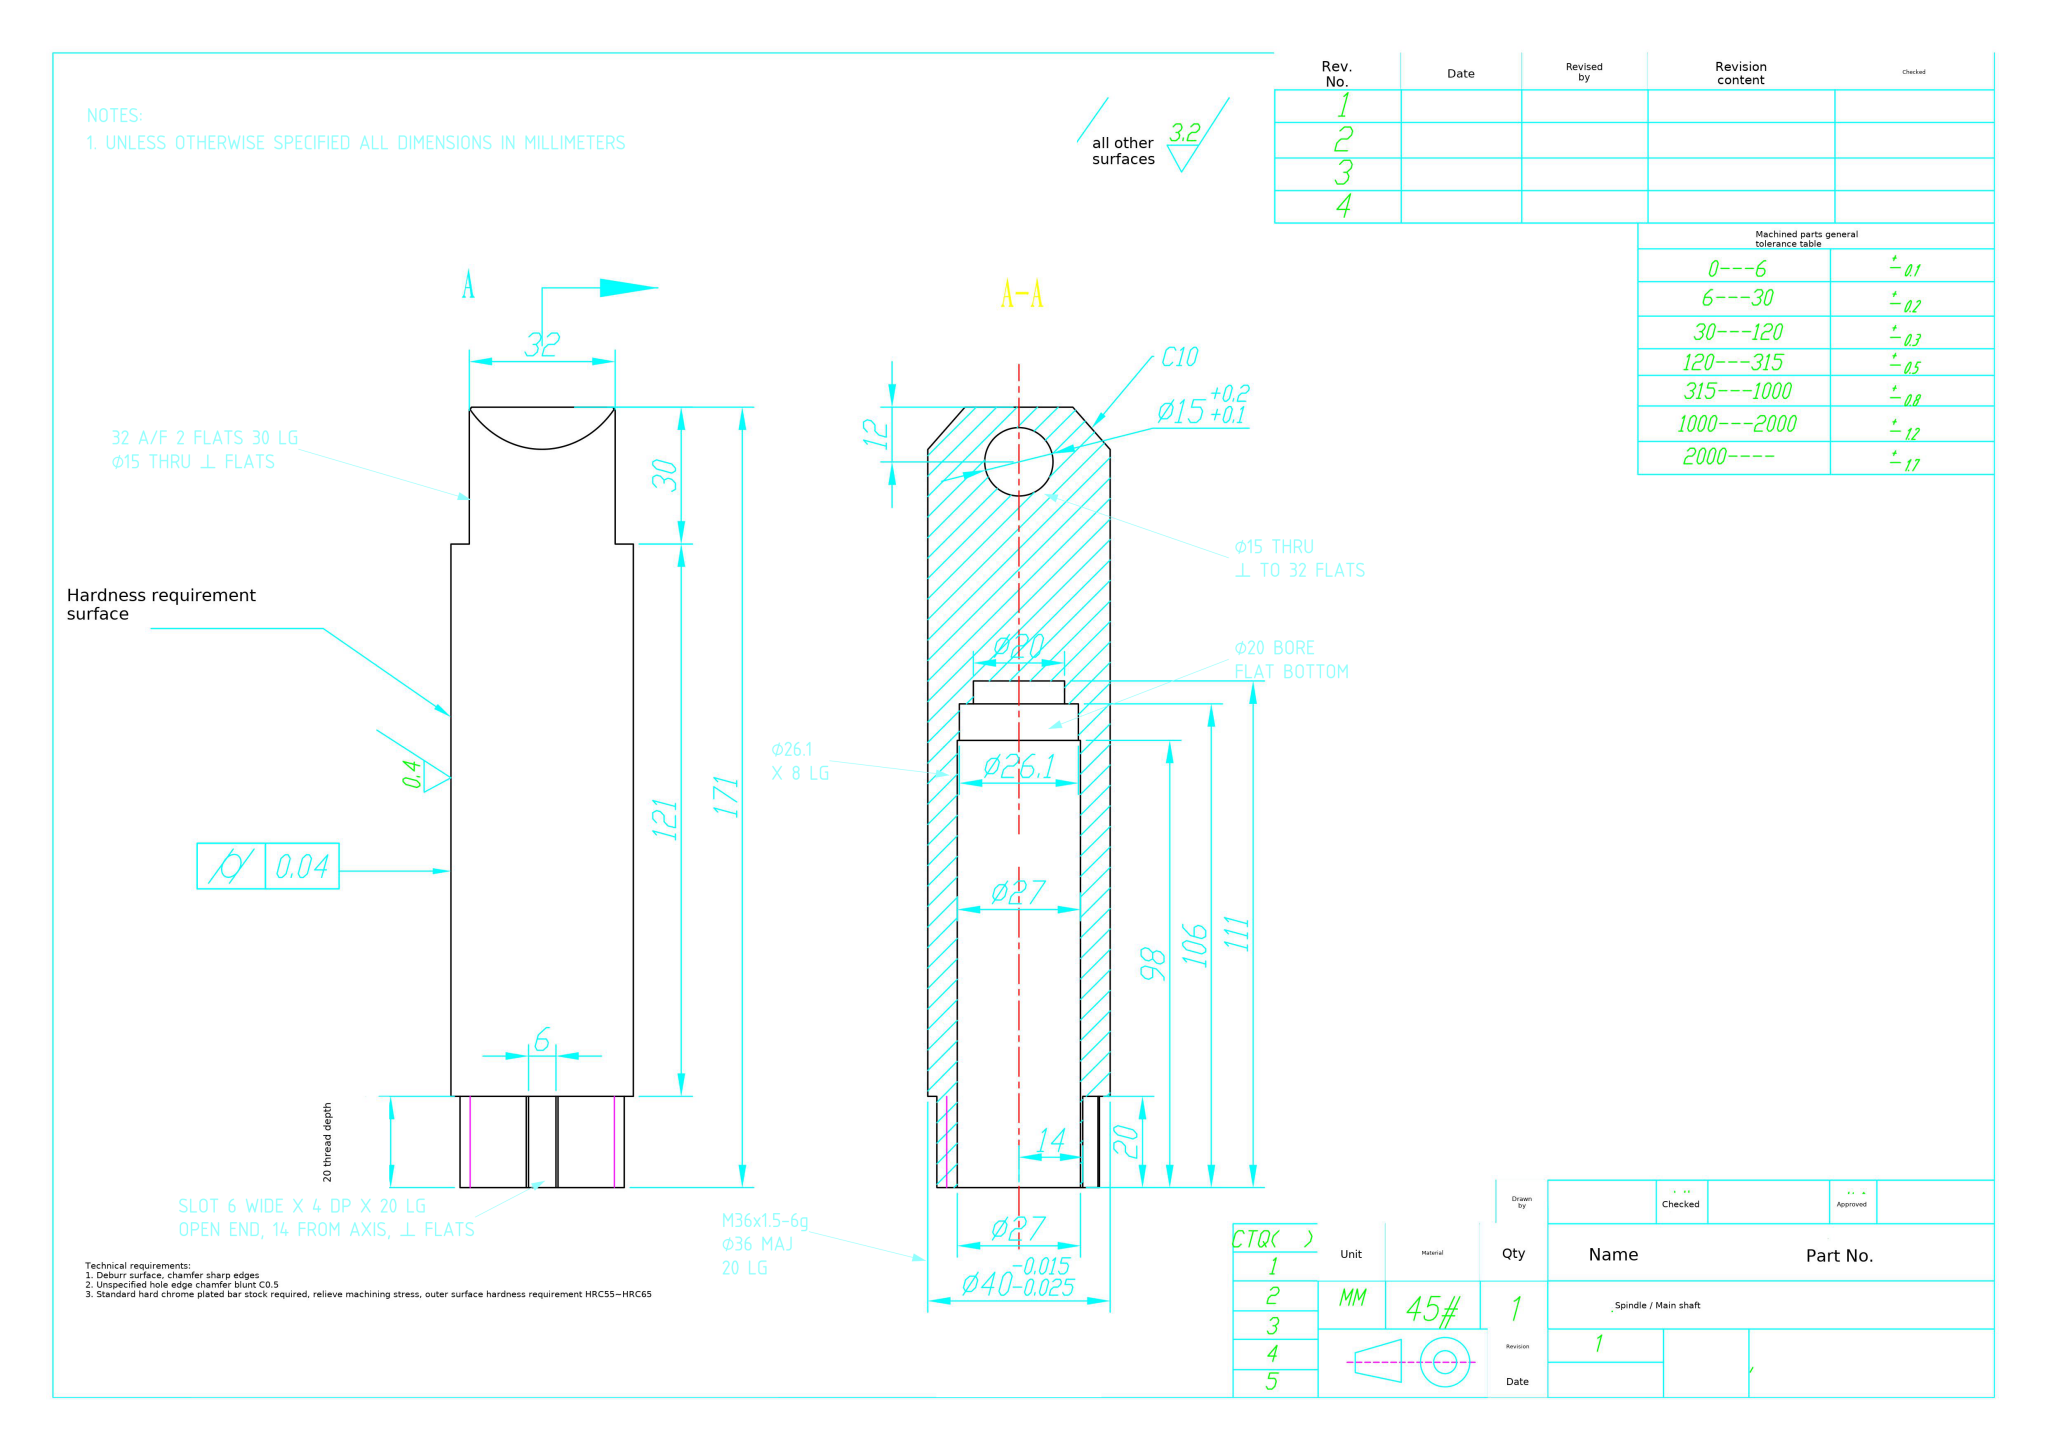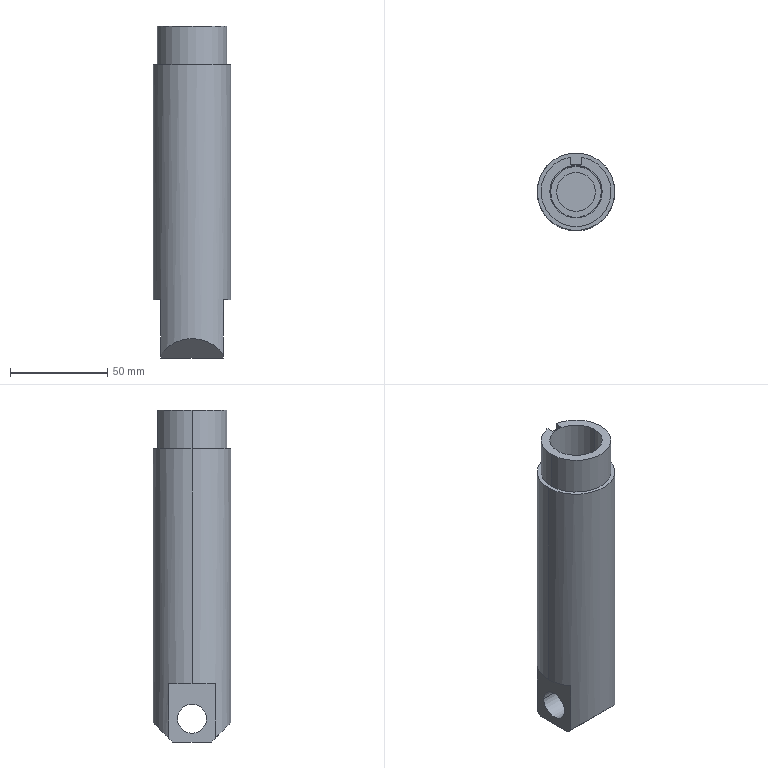Part | NX | mm | 1 solid | 30 faces | box 40 x 40 x 171 mm | volume 136084 mm3 | plane 17 | cylinder 13 | commonest cylinder face diameters 36 x3 40 x2 15 x2 20 x2 26.1 x2 27 x2
STEP:
#1=COLOUR_RGB('',0.7922,0.8196,0.9333);
#2=FILL_AREA_STYLE_COLOUR('',#1);
#3=FILL_AREA_STYLE('',(#2));
#4=SURFACE_STYLE_FILL_AREA(#3);
#5=SURFACE_SIDE_STYLE('',(#4));
#6=SURFACE_STYLE_USAGE(.BOTH.,#5);
#7=PRESENTATION_STYLE_ASSIGNMENT((#6));
#8=CARTESIAN_POINT('',(20.,0.,156.));
#9=VERTEX_POINT('',#8);
#10=CARTESIAN_POINT('',(-20.,0.,156.));
#11=VERTEX_POINT('',#10);
#12=CARTESIAN_POINT('',(0.,0.,156.));
#13=DIRECTION('',(0.,0.,1.));
#14=DIRECTION('',(1.,0.,0.));
#15=AXIS2_PLACEMENT_3D('',#12,#13,#14);
#16=CIRCLE('',#15,20.);
#17=EDGE_CURVE('',#9,#11,#16,.T.);
#18=ORIENTED_EDGE('',*,*,#17,.F.);
#19=CARTESIAN_POINT('',(20.,0.,35.));
#20=VERTEX_POINT('',#19);
#21=CARTESIAN_POINT('',(20.,0.,176.));
#22=DIRECTION('',(0.,0.,-1.));
#23=VECTOR('',#22,1000.);
#24=LINE('',#21,#23);
#25=EDGE_CURVE('',#9,#20,#24,.T.);
#26=ORIENTED_EDGE('',*,*,#25,.T.);
#27=CARTESIAN_POINT('',(16.,12.,35.));
#28=VERTEX_POINT('',#27);
#29=CARTESIAN_POINT('',(0.,0.,35.));
#30=DIRECTION('',(0.,0.,-1.));
#31=DIRECTION('',(-1.,0.,0.));
#32=AXIS2_PLACEMENT_3D('',#29,#30,#31);
#33=CIRCLE('',#32,20.);
#34=EDGE_CURVE('',#28,#20,#33,.T.);
#35=ORIENTED_EDGE('',*,*,#34,.F.);
#36=CARTESIAN_POINT('',(16.,12.,7.));
#37=VERTEX_POINT('',#36);
#38=CARTESIAN_POINT('',(16.,12.,176.));
#39=DIRECTION('',(0.,0.,-1.));
#40=VECTOR('',#39,1000.);
#41=LINE('',#38,#40);
#42=EDGE_CURVE('',#28,#37,#41,.T.);
#43=ORIENTED_EDGE('',*,*,#42,.T.);
#44=CARTESIAN_POINT('',(-16.,12.,7.));
#45=VERTEX_POINT('',#44);
#46=CARTESIAN_POINT('',(16.,12.,7.));
#47=CARTESIAN_POINT('',(7.273,23.636,18.636));
#48=CARTESIAN_POINT('',(-7.273,23.636,18.636));
#49=CARTESIAN_POINT('',(-16.,12.,7.));
#50=(BOUNDED_CURVE()B_SPLINE_CURVE(3,(#46,#47,#48,#49),.UNSPECIFIED.,.F.,.F.)B_SPLINE_CURVE_WITH_KNOTS((4,4),(2.214,4.069),.UNSPECIFIED.)CURVE()GEOMETRIC_REPRESENTATION_ITEM()RATIONAL_B_SPLINE_CURVE((1.,0.7333,0.7333,1.))REPRESENTATION_ITEM(''));
#51=EDGE_CURVE('',#37,#45,#50,.T.);
#52=ORIENTED_EDGE('',*,*,#51,.T.);
#53=CARTESIAN_POINT('',(-16.,12.,35.));
#54=VERTEX_POINT('',#53);
#55=CARTESIAN_POINT('',(-16.,12.,176.));
#56=DIRECTION('',(0.,0.,1.));
#57=VECTOR('',#56,1000.);
#58=LINE('',#55,#57);
#59=EDGE_CURVE('',#45,#54,#58,.T.);
#60=ORIENTED_EDGE('',*,*,#59,.T.);
#61=CARTESIAN_POINT('',(-20.,0.,35.));
#62=VERTEX_POINT('',#61);
#63=CARTESIAN_POINT('',(0.,0.,35.));
#64=DIRECTION('',(0.,0.,-1.));
#65=DIRECTION('',(-1.,0.,0.));
#66=AXIS2_PLACEMENT_3D('',#63,#64,#65);
#67=CIRCLE('',#66,20.);
#68=EDGE_CURVE('',#62,#54,#67,.T.);
#69=ORIENTED_EDGE('',*,*,#68,.F.);
#70=CARTESIAN_POINT('',(-20.,0.,176.));
#71=DIRECTION('',(0.,0.,-1.));
#72=VECTOR('',#71,1000.);
#73=LINE('',#70,#72);
#74=EDGE_CURVE('',#11,#62,#73,.T.);
#75=ORIENTED_EDGE('',*,*,#74,.F.);
#76=EDGE_LOOP('',(#18,#26,#35,#43,#52,#60,#69,#75));
#77=FACE_OUTER_BOUND('',#76,.T.);
#78=CARTESIAN_POINT('',(0.,0.,176.));
#79=DIRECTION('',(0.,0.,-1.));
#80=DIRECTION('',(-1.,0.,0.));
#81=AXIS2_PLACEMENT_3D('',#78,#79,#80);
#82=CYLINDRICAL_SURFACE('',#81,20.);
#83=ADVANCED_FACE('',(#77),#82,.T.);
#84=CARTESIAN_POINT('',(16.,7.5,17.));
#85=VERTEX_POINT('',#84);
#86=CARTESIAN_POINT('',(16.,-7.5,17.));
#87=VERTEX_POINT('',#86);
#88=CARTESIAN_POINT('',(16.,-0.,17.));
#89=DIRECTION('',(-1.,0.,0.));
#90=DIRECTION('',(0.,-1.,0.));
#91=AXIS2_PLACEMENT_3D('',#88,#89,#90);
#92=CIRCLE('',#91,7.5);
#93=EDGE_CURVE('',#85,#87,#92,.T.);
#94=ORIENTED_EDGE('',*,*,#93,.F.);
#95=CARTESIAN_POINT('',(-16.,7.5,17.));
#96=VERTEX_POINT('',#95);
#97=CARTESIAN_POINT('',(20.,7.5,17.));
#98=DIRECTION('',(-1.,0.,0.));
#99=VECTOR('',#98,1000.);
#100=LINE('',#97,#99);
#101=EDGE_CURVE('',#85,#96,#100,.T.);
#102=ORIENTED_EDGE('',*,*,#101,.T.);
#103=CARTESIAN_POINT('',(-16.,-7.5,17.));
#104=VERTEX_POINT('',#103);
#105=CARTESIAN_POINT('',(-16.,0.,17.));
#106=DIRECTION('',(-1.,0.,0.));
#107=DIRECTION('',(0.,-1.,0.));
#108=AXIS2_PLACEMENT_3D('',#105,#106,#107);
#109=CIRCLE('',#108,7.5);
#110=EDGE_CURVE('',#96,#104,#109,.T.);
#111=ORIENTED_EDGE('',*,*,#110,.T.);
#112=CARTESIAN_POINT('',(20.,-7.5,17.));
#113=DIRECTION('',(-1.,0.,0.));
#114=VECTOR('',#113,1000.);
#115=LINE('',#112,#114);
#116=EDGE_CURVE('',#87,#104,#115,.T.);
#117=ORIENTED_EDGE('',*,*,#116,.F.);
#118=EDGE_LOOP('',(#94,#102,#111,#117));
#119=FACE_OUTER_BOUND('',#118,.T.);
#120=CARTESIAN_POINT('',(20.,-0.,17.));
#121=DIRECTION('',(-1.,0.,0.));
#122=DIRECTION('',(0.,-1.,0.));
#123=AXIS2_PLACEMENT_3D('',#120,#121,#122);
#124=CYLINDRICAL_SURFACE('',#123,7.5);
#125=ADVANCED_FACE('',(#119),#124,.F.);
#126=CARTESIAN_POINT('',(-3.485,17.659,156.));
#127=VERTEX_POINT('',#126);
#128=CARTESIAN_POINT('',(-18.,0.,156.));
#129=VERTEX_POINT('',#128);
#130=CARTESIAN_POINT('',(0.,0.,156.));
#131=DIRECTION('',(0.,0.,1.));
#132=DIRECTION('',(1.,0.,0.));
#133=AXIS2_PLACEMENT_3D('',#130,#131,#132);
#134=CIRCLE('',#133,18.);
#135=EDGE_CURVE('',#127,#129,#134,.T.);
#136=ORIENTED_EDGE('',*,*,#135,.T.);
#137=CARTESIAN_POINT('',(-18.,0.,176.));
#138=VERTEX_POINT('',#137);
#139=CARTESIAN_POINT('',(-18.,0.,156.));
#140=DIRECTION('',(0.,0.,1.));
#141=VECTOR('',#140,1000.);
#142=LINE('',#139,#141);
#143=EDGE_CURVE('',#129,#138,#142,.T.);
#144=ORIENTED_EDGE('',*,*,#143,.T.);
#145=CARTESIAN_POINT('',(-3.485,17.659,176.));
#146=VERTEX_POINT('',#145);
#147=CARTESIAN_POINT('',(0.,0.,176.));
#148=DIRECTION('',(0.,0.,1.));
#149=DIRECTION('',(1.,0.,0.));
#150=AXIS2_PLACEMENT_3D('',#147,#148,#149);
#151=CIRCLE('',#150,18.);
#152=EDGE_CURVE('',#146,#138,#151,.T.);
#153=ORIENTED_EDGE('',*,*,#152,.F.);
#154=CARTESIAN_POINT('',(-3.485,17.659,156.));
#155=DIRECTION('',(0.,0.,-1.));
#156=VECTOR('',#155,1000.);
#157=LINE('',#154,#156);
#158=EDGE_CURVE('',#146,#127,#157,.T.);
#159=ORIENTED_EDGE('',*,*,#158,.T.);
#160=EDGE_LOOP('',(#136,#144,#153,#159));
#161=FACE_OUTER_BOUND('',#160,.T.);
#162=CARTESIAN_POINT('',(0.,0.,156.));
#163=DIRECTION('',(0.,0.,1.));
#164=DIRECTION('',(1.,0.,0.));
#165=AXIS2_PLACEMENT_3D('',#162,#163,#164);
#166=CYLINDRICAL_SURFACE('',#165,18.);
#167=ADVANCED_FACE('',(#161),#166,.T.);
#168=ORIENTED_EDGE('',*,*,#143,.F.);
#169=CARTESIAN_POINT('',(18.,0.,156.));
#170=VERTEX_POINT('',#169);
#171=CARTESIAN_POINT('',(0.,0.,156.));
#172=DIRECTION('',(0.,0.,1.));
#173=DIRECTION('',(1.,0.,0.));
#174=AXIS2_PLACEMENT_3D('',#171,#172,#173);
#175=CIRCLE('',#174,18.);
#176=EDGE_CURVE('',#129,#170,#175,.T.);
#177=ORIENTED_EDGE('',*,*,#176,.T.);
#178=CARTESIAN_POINT('',(18.,0.,176.));
#179=VERTEX_POINT('',#178);
#180=CARTESIAN_POINT('',(18.,0.,156.));
#181=DIRECTION('',(0.,0.,1.));
#182=VECTOR('',#181,1000.);
#183=LINE('',#180,#182);
#184=EDGE_CURVE('',#170,#179,#183,.T.);
#185=ORIENTED_EDGE('',*,*,#184,.T.);
#186=CARTESIAN_POINT('',(0.,0.,176.));
#187=DIRECTION('',(0.,0.,1.));
#188=DIRECTION('',(1.,0.,0.));
#189=AXIS2_PLACEMENT_3D('',#186,#187,#188);
#190=CIRCLE('',#189,18.);
#191=EDGE_CURVE('',#138,#179,#190,.T.);
#192=ORIENTED_EDGE('',*,*,#191,.F.);
#193=EDGE_LOOP('',(#168,#177,#185,#192));
#194=FACE_OUTER_BOUND('',#193,.T.);
#195=CARTESIAN_POINT('',(0.,0.,156.));
#196=DIRECTION('',(0.,0.,1.));
#197=DIRECTION('',(1.,0.,0.));
#198=AXIS2_PLACEMENT_3D('',#195,#196,#197);
#199=CYLINDRICAL_SURFACE('',#198,18.);
#200=ADVANCED_FACE('',(#194),#199,.T.);
#201=CARTESIAN_POINT('',(-10.,0.,65.));
#202=VERTEX_POINT('',#201);
#203=CARTESIAN_POINT('',(10.,0.,65.));
#204=VERTEX_POINT('',#203);
#205=CARTESIAN_POINT('',(0.,0.,65.));
#206=DIRECTION('',(0.,0.,1.));
#207=DIRECTION('',(1.,0.,0.));
#208=AXIS2_PLACEMENT_3D('',#205,#206,#207);
#209=CIRCLE('',#208,10.);
#210=EDGE_CURVE('',#202,#204,#209,.T.);
#211=ORIENTED_EDGE('',*,*,#210,.F.);
#212=CARTESIAN_POINT('',(-10.,0.,70.));
#213=VERTEX_POINT('',#212);
#214=CARTESIAN_POINT('',(-10.,0.,65.));
#215=DIRECTION('',(0.,0.,1.));
#216=VECTOR('',#215,1000.);
#217=LINE('',#214,#216);
#218=EDGE_CURVE('',#202,#213,#217,.T.);
#219=ORIENTED_EDGE('',*,*,#218,.T.);
#220=CARTESIAN_POINT('',(10.,0.,70.));
#221=VERTEX_POINT('',#220);
#222=CARTESIAN_POINT('',(0.,0.,70.));
#223=DIRECTION('',(0.,0.,1.));
#224=DIRECTION('',(1.,0.,0.));
#225=AXIS2_PLACEMENT_3D('',#222,#223,#224);
#226=CIRCLE('',#225,10.);
#227=EDGE_CURVE('',#213,#221,#226,.T.);
#228=ORIENTED_EDGE('',*,*,#227,.T.);
#229=CARTESIAN_POINT('',(10.,0.,65.));
#230=DIRECTION('',(0.,0.,1.));
#231=VECTOR('',#230,1000.);
#232=LINE('',#229,#231);
#233=EDGE_CURVE('',#204,#221,#232,.T.);
#234=ORIENTED_EDGE('',*,*,#233,.F.);
#235=EDGE_LOOP('',(#211,#219,#228,#234));
#236=FACE_OUTER_BOUND('',#235,.T.);
#237=CARTESIAN_POINT('',(0.,0.,65.));
#238=DIRECTION('',(0.,0.,1.));
#239=DIRECTION('',(1.,0.,0.));
#240=AXIS2_PLACEMENT_3D('',#237,#238,#239);
#241=CYLINDRICAL_SURFACE('',#240,10.);
#242=ADVANCED_FACE('',(#236),#241,.F.);
#243=CARTESIAN_POINT('',(-13.05,0.,70.));
#244=VERTEX_POINT('',#243);
#245=CARTESIAN_POINT('',(13.05,0.,70.));
#246=VERTEX_POINT('',#245);
#247=CARTESIAN_POINT('',(0.,0.,70.));
#248=DIRECTION('',(0.,0.,1.));
#249=DIRECTION('',(1.,0.,0.));
#250=AXIS2_PLACEMENT_3D('',#247,#248,#249);
#251=CIRCLE('',#250,13.05);
#252=EDGE_CURVE('',#244,#246,#251,.T.);
#253=ORIENTED_EDGE('',*,*,#252,.F.);
#254=CARTESIAN_POINT('',(-13.05,0.,78.));
#255=VERTEX_POINT('',#254);
#256=CARTESIAN_POINT('',(-13.05,0.,70.));
#257=DIRECTION('',(0.,0.,1.));
#258=VECTOR('',#257,1000.);
#259=LINE('',#256,#258);
#260=EDGE_CURVE('',#244,#255,#259,.T.);
#261=ORIENTED_EDGE('',*,*,#260,.T.);
#262=CARTESIAN_POINT('',(13.05,0.,78.));
#263=VERTEX_POINT('',#262);
#264=CARTESIAN_POINT('',(0.,0.,78.));
#265=DIRECTION('',(0.,0.,1.));
#266=DIRECTION('',(1.,0.,0.));
#267=AXIS2_PLACEMENT_3D('',#264,#265,#266);
#268=CIRCLE('',#267,13.05);
#269=EDGE_CURVE('',#255,#263,#268,.T.);
#270=ORIENTED_EDGE('',*,*,#269,.T.);
#271=CARTESIAN_POINT('',(13.05,0.,70.));
#272=DIRECTION('',(0.,0.,1.));
#273=VECTOR('',#272,1000.);
#274=LINE('',#271,#273);
#275=EDGE_CURVE('',#246,#263,#274,.T.);
#276=ORIENTED_EDGE('',*,*,#275,.F.);
#277=EDGE_LOOP('',(#253,#261,#270,#276));
#278=FACE_OUTER_BOUND('',#277,.T.);
#279=CARTESIAN_POINT('',(0.,0.,70.));
#280=DIRECTION('',(0.,0.,1.));
#281=DIRECTION('',(1.,0.,0.));
#282=AXIS2_PLACEMENT_3D('',#279,#280,#281);
#283=CYLINDRICAL_SURFACE('',#282,13.05);
#284=ADVANCED_FACE('',(#278),#283,.F.);
#285=CARTESIAN_POINT('',(-13.5,0.,78.));
#286=VERTEX_POINT('',#285);
#287=CARTESIAN_POINT('',(13.5,0.,78.));
#288=VERTEX_POINT('',#287);
#289=CARTESIAN_POINT('',(0.,0.,78.));
#290=DIRECTION('',(0.,0.,1.));
#291=DIRECTION('',(1.,0.,0.));
#292=AXIS2_PLACEMENT_3D('',#289,#290,#291);
#293=CIRCLE('',#292,13.5);
#294=EDGE_CURVE('',#286,#288,#293,.T.);
#295=ORIENTED_EDGE('',*,*,#294,.F.);
#296=CARTESIAN_POINT('',(-13.5,0.,176.));
#297=VERTEX_POINT('',#296);
#298=CARTESIAN_POINT('',(-13.5,0.,78.));
#299=DIRECTION('',(0.,0.,1.));
#300=VECTOR('',#299,1000.);
#301=LINE('',#298,#300);
#302=EDGE_CURVE('',#286,#297,#301,.T.);
#303=ORIENTED_EDGE('',*,*,#302,.T.);
#304=CARTESIAN_POINT('',(13.5,0.,176.));
#305=VERTEX_POINT('',#304);
#306=CARTESIAN_POINT('',(0.,0.,176.));
#307=DIRECTION('',(0.,0.,1.));
#308=DIRECTION('',(1.,0.,0.));
#309=AXIS2_PLACEMENT_3D('',#306,#307,#308);
#310=CIRCLE('',#309,13.5);
#311=EDGE_CURVE('',#297,#305,#310,.T.);
#312=ORIENTED_EDGE('',*,*,#311,.T.);
#313=CARTESIAN_POINT('',(13.5,0.,78.));
#314=DIRECTION('',(0.,0.,1.));
#315=VECTOR('',#314,1000.);
#316=LINE('',#313,#315);
#317=EDGE_CURVE('',#288,#305,#316,.T.);
#318=ORIENTED_EDGE('',*,*,#317,.F.);
#319=EDGE_LOOP('',(#295,#303,#312,#318));
#320=FACE_OUTER_BOUND('',#319,.T.);
#321=CARTESIAN_POINT('',(0.,0.,78.));
#322=DIRECTION('',(0.,0.,1.));
#323=DIRECTION('',(1.,0.,0.));
#324=AXIS2_PLACEMENT_3D('',#321,#322,#323);
#325=CYLINDRICAL_SURFACE('',#324,13.5);
#326=ADVANCED_FACE('',(#320),#325,.F.);
#327=ORIENTED_EDGE('',*,*,#152,.T.);
#328=ORIENTED_EDGE('',*,*,#191,.T.);
#329=CARTESIAN_POINT('',(3.485,17.659,176.));
#330=VERTEX_POINT('',#329);
#331=CARTESIAN_POINT('',(0.,0.,176.));
#332=DIRECTION('',(0.,0.,1.));
#333=DIRECTION('',(1.,0.,0.));
#334=AXIS2_PLACEMENT_3D('',#331,#332,#333);
#335=CIRCLE('',#334,18.);
#336=EDGE_CURVE('',#179,#330,#335,.T.);
#337=ORIENTED_EDGE('',*,*,#336,.T.);
#338=CARTESIAN_POINT('',(3.,17.314,176.));
#339=VERTEX_POINT('',#338);
#340=CARTESIAN_POINT('',(-7.169,10.086,176.));
#341=DIRECTION('',(-0.8151,-0.5794,0.));
#342=VECTOR('',#341,1000.);
#343=LINE('',#340,#342);
#344=EDGE_CURVE('',#330,#339,#343,.T.);
#345=ORIENTED_EDGE('',*,*,#344,.T.);
#346=CARTESIAN_POINT('',(3.,14.,176.));
#347=VERTEX_POINT('',#346);
#348=CARTESIAN_POINT('',(3.,18.886,176.));
#349=DIRECTION('',(-0.,1.,0.));
#350=VECTOR('',#349,1000.);
#351=LINE('',#348,#350);
#352=EDGE_CURVE('',#347,#339,#351,.T.);
#353=ORIENTED_EDGE('',*,*,#352,.F.);
#354=CARTESIAN_POINT('',(-3.,14.,176.));
#355=VERTEX_POINT('',#354);
#356=CARTESIAN_POINT('',(-3.,14.,176.));
#357=DIRECTION('',(1.,0.,0.));
#358=VECTOR('',#357,1000.);
#359=LINE('',#356,#358);
#360=EDGE_CURVE('',#355,#347,#359,.T.);
#361=ORIENTED_EDGE('',*,*,#360,.F.);
#362=CARTESIAN_POINT('',(-3.,17.314,176.));
#363=VERTEX_POINT('',#362);
#364=CARTESIAN_POINT('',(-3.,18.886,176.));
#365=DIRECTION('',(0.,-1.,0.));
#366=VECTOR('',#365,1000.);
#367=LINE('',#364,#366);
#368=EDGE_CURVE('',#363,#355,#367,.T.);
#369=ORIENTED_EDGE('',*,*,#368,.F.);
#370=CARTESIAN_POINT('',(7.169,10.086,176.));
#371=DIRECTION('',(-0.8151,0.5794,0.));
#372=VECTOR('',#371,1000.);
#373=LINE('',#370,#372);
#374=EDGE_CURVE('',#363,#146,#373,.T.);
#375=ORIENTED_EDGE('',*,*,#374,.T.);
#376=EDGE_LOOP('',(#327,#328,#337,#345,#353,#361,#369,#375));
#377=FACE_OUTER_BOUND('',#376,.T.);
#378=CARTESIAN_POINT('',(0.,0.,176.));
#379=DIRECTION('',(0.,0.,1.));
#380=DIRECTION('',(1.,0.,0.));
#381=AXIS2_PLACEMENT_3D('',#378,#379,#380);
#382=CIRCLE('',#381,13.5);
#383=EDGE_CURVE('',#305,#297,#382,.T.);
#384=ORIENTED_EDGE('',*,*,#383,.F.);
#385=ORIENTED_EDGE('',*,*,#311,.F.);
#386=EDGE_LOOP('',(#384,#385));
#387=FACE_BOUND('',#386,.T.);
#388=CARTESIAN_POINT('',(0.,0.,176.));
#389=DIRECTION('',(0.,0.,1.));
#390=DIRECTION('',(1.,0.,0.));
#391=AXIS2_PLACEMENT_3D('',#388,#389,#390);
#392=PLANE('',#391);
#393=ADVANCED_FACE('',(#377,#387),#392,.T.);
#394=ORIENTED_EDGE('',*,*,#302,.F.);
#395=CARTESIAN_POINT('',(0.,0.,78.));
#396=DIRECTION('',(0.,0.,1.));
#397=DIRECTION('',(1.,0.,0.));
#398=AXIS2_PLACEMENT_3D('',#395,#396,#397);
#399=CIRCLE('',#398,13.5);
#400=EDGE_CURVE('',#288,#286,#399,.T.);
#401=ORIENTED_EDGE('',*,*,#400,.F.);
#402=ORIENTED_EDGE('',*,*,#317,.T.);
#403=ORIENTED_EDGE('',*,*,#383,.T.);
#404=EDGE_LOOP('',(#394,#401,#402,#403));
#405=FACE_OUTER_BOUND('',#404,.T.);
#406=CARTESIAN_POINT('',(0.,0.,78.));
#407=DIRECTION('',(0.,0.,1.));
#408=DIRECTION('',(1.,0.,0.));
#409=AXIS2_PLACEMENT_3D('',#406,#407,#408);
#410=CYLINDRICAL_SURFACE('',#409,13.5);
#411=ADVANCED_FACE('',(#405),#410,.F.);
#412=CARTESIAN_POINT('',(0.,0.,78.));
#413=DIRECTION('',(0.,0.,1.));
#414=DIRECTION('',(1.,0.,0.));
#415=AXIS2_PLACEMENT_3D('',#412,#413,#414);
#416=CIRCLE('',#415,13.05);
#417=EDGE_CURVE('',#263,#255,#416,.T.);
#418=ORIENTED_EDGE('',*,*,#417,.F.);
#419=ORIENTED_EDGE('',*,*,#269,.F.);
#420=EDGE_LOOP('',(#418,#419));
#421=FACE_BOUND('',#420,.T.);
#422=ORIENTED_EDGE('',*,*,#400,.T.);
#423=ORIENTED_EDGE('',*,*,#294,.T.);
#424=EDGE_LOOP('',(#422,#423));
#425=FACE_OUTER_BOUND('',#424,.T.);
#426=CARTESIAN_POINT('',(0.,0.,78.));
#427=DIRECTION('',(0.,0.,1.));
#428=DIRECTION('',(1.,0.,0.));
#429=AXIS2_PLACEMENT_3D('',#426,#427,#428);
#430=PLANE('',#429);
#431=ADVANCED_FACE('',(#421,#425),#430,.T.);
#432=ORIENTED_EDGE('',*,*,#260,.F.);
#433=CARTESIAN_POINT('',(0.,0.,70.));
#434=DIRECTION('',(0.,0.,1.));
#435=DIRECTION('',(1.,0.,0.));
#436=AXIS2_PLACEMENT_3D('',#433,#434,#435);
#437=CIRCLE('',#436,13.05);
#438=EDGE_CURVE('',#246,#244,#437,.T.);
#439=ORIENTED_EDGE('',*,*,#438,.F.);
#440=ORIENTED_EDGE('',*,*,#275,.T.);
#441=ORIENTED_EDGE('',*,*,#417,.T.);
#442=EDGE_LOOP('',(#432,#439,#440,#441));
#443=FACE_OUTER_BOUND('',#442,.T.);
#444=CARTESIAN_POINT('',(0.,0.,70.));
#445=DIRECTION('',(0.,0.,1.));
#446=DIRECTION('',(1.,0.,0.));
#447=AXIS2_PLACEMENT_3D('',#444,#445,#446);
#448=CYLINDRICAL_SURFACE('',#447,13.05);
#449=ADVANCED_FACE('',(#443),#448,.F.);
#450=CARTESIAN_POINT('',(0.,0.,70.));
#451=DIRECTION('',(0.,0.,1.));
#452=DIRECTION('',(1.,0.,0.));
#453=AXIS2_PLACEMENT_3D('',#450,#451,#452);
#454=CIRCLE('',#453,10.);
#455=EDGE_CURVE('',#221,#213,#454,.T.);
#456=ORIENTED_EDGE('',*,*,#455,.F.);
#457=ORIENTED_EDGE('',*,*,#227,.F.);
#458=EDGE_LOOP('',(#456,#457));
#459=FACE_BOUND('',#458,.T.);
#460=ORIENTED_EDGE('',*,*,#438,.T.);
#461=ORIENTED_EDGE('',*,*,#252,.T.);
#462=EDGE_LOOP('',(#460,#461));
#463=FACE_OUTER_BOUND('',#462,.T.);
#464=CARTESIAN_POINT('',(0.,0.,70.));
#465=DIRECTION('',(0.,0.,1.));
#466=DIRECTION('',(1.,0.,0.));
#467=AXIS2_PLACEMENT_3D('',#464,#465,#466);
#468=PLANE('',#467);
#469=ADVANCED_FACE('',(#459,#463),#468,.T.);
#470=ORIENTED_EDGE('',*,*,#218,.F.);
#471=CARTESIAN_POINT('',(0.,0.,65.));
#472=DIRECTION('',(0.,0.,1.));
#473=DIRECTION('',(1.,0.,0.));
#474=AXIS2_PLACEMENT_3D('',#471,#472,#473);
#475=CIRCLE('',#474,10.);
#476=EDGE_CURVE('',#204,#202,#475,.T.);
#477=ORIENTED_EDGE('',*,*,#476,.F.);
#478=ORIENTED_EDGE('',*,*,#233,.T.);
#479=ORIENTED_EDGE('',*,*,#455,.T.);
#480=EDGE_LOOP('',(#470,#477,#478,#479));
#481=FACE_OUTER_BOUND('',#480,.T.);
#482=CARTESIAN_POINT('',(0.,0.,65.));
#483=DIRECTION('',(0.,0.,1.));
#484=DIRECTION('',(1.,0.,0.));
#485=AXIS2_PLACEMENT_3D('',#482,#483,#484);
#486=CYLINDRICAL_SURFACE('',#485,10.);
#487=ADVANCED_FACE('',(#481),#486,.F.);
#488=ORIENTED_EDGE('',*,*,#476,.T.);
#489=ORIENTED_EDGE('',*,*,#210,.T.);
#490=EDGE_LOOP('',(#488,#489));
#491=FACE_OUTER_BOUND('',#490,.T.);
#492=CARTESIAN_POINT('',(0.,0.,65.));
#493=DIRECTION('',(0.,0.,1.));
#494=DIRECTION('',(1.,0.,0.));
#495=AXIS2_PLACEMENT_3D('',#492,#493,#494);
#496=PLANE('',#495);
#497=ADVANCED_FACE('',(#491),#496,.T.);
#498=ORIENTED_EDGE('',*,*,#135,.F.);
#499=CARTESIAN_POINT('',(-3.,17.314,156.));
#500=VERTEX_POINT('',#499);
#501=CARTESIAN_POINT('',(-3.,17.314,156.));
#502=DIRECTION('',(0.8151,-0.5794,0.));
#503=VECTOR('',#502,1000.);
#504=LINE('',#501,#503);
#505=EDGE_CURVE('',#127,#500,#504,.T.);
#506=ORIENTED_EDGE('',*,*,#505,.T.);
#507=CARTESIAN_POINT('',(-3.,14.,156.));
#508=VERTEX_POINT('',#507);
#509=CARTESIAN_POINT('',(-3.,18.886,156.));
#510=DIRECTION('',(-0.,1.,0.));
#511=VECTOR('',#510,1000.);
#512=LINE('',#509,#511);
#513=EDGE_CURVE('',#508,#500,#512,.T.);
#514=ORIENTED_EDGE('',*,*,#513,.F.);
#515=CARTESIAN_POINT('',(3.,14.,156.));
#516=VERTEX_POINT('',#515);
#517=CARTESIAN_POINT('',(-3.,14.,156.));
#518=DIRECTION('',(-1.,0.,0.));
#519=VECTOR('',#518,1000.);
#520=LINE('',#517,#519);
#521=EDGE_CURVE('',#516,#508,#520,.T.);
#522=ORIENTED_EDGE('',*,*,#521,.F.);
#523=CARTESIAN_POINT('',(3.,17.314,156.));
#524=VERTEX_POINT('',#523);
#525=CARTESIAN_POINT('',(3.,18.886,156.));
#526=DIRECTION('',(0.,-1.,0.));
#527=VECTOR('',#526,1000.);
#528=LINE('',#525,#527);
#529=EDGE_CURVE('',#524,#516,#528,.T.);
#530=ORIENTED_EDGE('',*,*,#529,.F.);
#531=CARTESIAN_POINT('',(3.485,17.659,156.));
#532=VERTEX_POINT('',#531);
#533=CARTESIAN_POINT('',(3.,17.314,156.));
#534=DIRECTION('',(0.8151,0.5794,0.));
#535=VECTOR('',#534,1000.);
#536=LINE('',#533,#535);
#537=EDGE_CURVE('',#524,#532,#536,.T.);
#538=ORIENTED_EDGE('',*,*,#537,.T.);
#539=CARTESIAN_POINT('',(0.,0.,156.));
#540=DIRECTION('',(0.,0.,1.));
#541=DIRECTION('',(1.,0.,0.));
#542=AXIS2_PLACEMENT_3D('',#539,#540,#541);
#543=CIRCLE('',#542,18.);
#544=EDGE_CURVE('',#170,#532,#543,.T.);
#545=ORIENTED_EDGE('',*,*,#544,.F.);
#546=ORIENTED_EDGE('',*,*,#176,.F.);
#547=EDGE_LOOP('',(#498,#506,#514,#522,#530,#538,#545,#546));
#548=FACE_BOUND('',#547,.T.);
#549=CARTESIAN_POINT('',(0.,0.,156.));
#550=DIRECTION('',(0.,0.,1.));
#551=DIRECTION('',(1.,0.,0.));
#552=AXIS2_PLACEMENT_3D('',#549,#550,#551);
#553=CIRCLE('',#552,20.);
#554=EDGE_CURVE('',#11,#9,#553,.T.);
#555=ORIENTED_EDGE('',*,*,#554,.T.);
#556=ORIENTED_EDGE('',*,*,#17,.T.);
#557=EDGE_LOOP('',(#555,#556));
#558=FACE_OUTER_BOUND('',#557,.T.);
#559=CARTESIAN_POINT('',(0.,0.,156.));
#560=DIRECTION('',(0.,0.,1.));
#561=DIRECTION('',(1.,0.,0.));
#562=AXIS2_PLACEMENT_3D('',#559,#560,#561);
#563=PLANE('',#562);
#564=ADVANCED_FACE('',(#548,#558),#563,.T.);
#565=ORIENTED_EDGE('',*,*,#184,.F.);
#566=ORIENTED_EDGE('',*,*,#544,.T.);
#567=CARTESIAN_POINT('',(3.485,17.659,156.));
#568=DIRECTION('',(0.,0.,1.));
#569=VECTOR('',#568,1000.);
#570=LINE('',#567,#569);
#571=EDGE_CURVE('',#532,#330,#570,.T.);
#572=ORIENTED_EDGE('',*,*,#571,.T.);
#573=ORIENTED_EDGE('',*,*,#336,.F.);
#574=EDGE_LOOP('',(#565,#566,#572,#573));
#575=FACE_OUTER_BOUND('',#574,.T.);
#576=CARTESIAN_POINT('',(0.,0.,156.));
#577=DIRECTION('',(0.,0.,1.));
#578=DIRECTION('',(1.,0.,0.));
#579=AXIS2_PLACEMENT_3D('',#576,#577,#578);
#580=CYLINDRICAL_SURFACE('',#579,18.);
#581=ADVANCED_FACE('',(#575),#580,.T.);
#582=ORIENTED_EDGE('',*,*,#101,.F.);
#583=CARTESIAN_POINT('',(16.,-0.,17.));
#584=DIRECTION('',(-1.,0.,0.));
#585=DIRECTION('',(0.,-1.,0.));
#586=AXIS2_PLACEMENT_3D('',#583,#584,#585);
#587=CIRCLE('',#586,7.5);
#588=EDGE_CURVE('',#87,#85,#587,.T.);
#589=ORIENTED_EDGE('',*,*,#588,.F.);
#590=ORIENTED_EDGE('',*,*,#116,.T.);
#591=CARTESIAN_POINT('',(-16.,0.,17.));
#592=DIRECTION('',(-1.,0.,0.));
#593=DIRECTION('',(0.,-1.,0.));
#594=AXIS2_PLACEMENT_3D('',#591,#592,#593);
#595=CIRCLE('',#594,7.5);
#596=EDGE_CURVE('',#104,#96,#595,.T.);
#597=ORIENTED_EDGE('',*,*,#596,.T.);
#598=EDGE_LOOP('',(#582,#589,#590,#597));
#599=FACE_OUTER_BOUND('',#598,.T.);
#600=CARTESIAN_POINT('',(20.,-0.,17.));
#601=DIRECTION('',(-1.,0.,0.));
#602=DIRECTION('',(0.,-1.,0.));
#603=AXIS2_PLACEMENT_3D('',#600,#601,#602);
#604=CYLINDRICAL_SURFACE('',#603,7.5);
#605=ADVANCED_FACE('',(#599),#604,.F.);
#606=CARTESIAN_POINT('',(-16.,-12.,35.));
#607=VERTEX_POINT('',#606);
#608=CARTESIAN_POINT('',(0.,0.,35.));
#609=DIRECTION('',(0.,0.,-1.));
#610=DIRECTION('',(-1.,0.,0.));
#611=AXIS2_PLACEMENT_3D('',#608,#609,#610);
#612=CIRCLE('',#611,20.);
#613=EDGE_CURVE('',#607,#62,#612,.T.);
#614=ORIENTED_EDGE('',*,*,#613,.T.);
#615=ORIENTED_EDGE('',*,*,#68,.T.);
#616=CARTESIAN_POINT('',(-16.,18.975,35.));
#617=DIRECTION('',(-0.,-1.,0.));
#618=VECTOR('',#617,1000.);
#619=LINE('',#616,#618);
#620=EDGE_CURVE('',#54,#607,#619,.T.);
#621=ORIENTED_EDGE('',*,*,#620,.T.);
#622=EDGE_LOOP('',(#614,#615,#621));
#623=FACE_OUTER_BOUND('',#622,.T.);
#624=CARTESIAN_POINT('',(0.,0.,35.));
#625=DIRECTION('',(0.,0.,-1.));
#626=DIRECTION('',(-1.,0.,0.));
#627=AXIS2_PLACEMENT_3D('',#624,#625,#626);
#628=PLANE('',#627);
#629=ADVANCED_FACE('',(#623),#628,.T.);
#630=ORIENTED_EDGE('',*,*,#34,.T.);
#631=CARTESIAN_POINT('',(16.,-12.,35.));
#632=VERTEX_POINT('',#631);
#633=CARTESIAN_POINT('',(0.,0.,35.));
#634=DIRECTION('',(0.,0.,-1.));
#635=DIRECTION('',(-1.,0.,0.));
#636=AXIS2_PLACEMENT_3D('',#633,#634,#635);
#637=CIRCLE('',#636,20.);
#638=EDGE_CURVE('',#20,#632,#637,.T.);
#639=ORIENTED_EDGE('',*,*,#638,.T.);
#640=CARTESIAN_POINT('',(16.,18.975,35.));
#641=DIRECTION('',(0.,1.,0.));
#642=VECTOR('',#641,1000.);
#643=LINE('',#640,#642);
#644=EDGE_CURVE('',#632,#28,#643,.T.);
#645=ORIENTED_EDGE('',*,*,#644,.T.);
#646=EDGE_LOOP('',(#630,#639,#645));
#647=FACE_OUTER_BOUND('',#646,.T.);
#648=CARTESIAN_POINT('',(0.,0.,35.));
#649=DIRECTION('',(0.,0.,-1.));
#650=DIRECTION('',(-1.,0.,0.));
#651=AXIS2_PLACEMENT_3D('',#648,#649,#650);
#652=PLANE('',#651);
#653=ADVANCED_FACE('',(#647),#652,.T.);
#654=ORIENTED_EDGE('',*,*,#588,.T.);
#655=ORIENTED_EDGE('',*,*,#93,.T.);
#656=EDGE_LOOP('',(#654,#655));
#657=FACE_BOUND('',#656,.T.);
#658=CARTESIAN_POINT('',(16.,10.,5.));
#659=VERTEX_POINT('',#658);
#660=CARTESIAN_POINT('',(16.,-10.,5.));
#661=VERTEX_POINT('',#660);
#662=CARTESIAN_POINT('',(16.,22.744,5.));
#663=DIRECTION('',(-0.,-1.,-0.));
#664=VECTOR('',#663,1000.);
#665=LINE('',#662,#664);
#666=EDGE_CURVE('',#659,#661,#665,.T.);
#667=ORIENTED_EDGE('',*,*,#666,.F.);
#668=CARTESIAN_POINT('',(16.,10.,5.));
#669=DIRECTION('',(0.,-0.7071,-0.7071));
#670=VECTOR('',#669,1000.);
#671=LINE('',#668,#670);
#672=EDGE_CURVE('',#37,#659,#671,.T.);
#673=ORIENTED_EDGE('',*,*,#672,.F.);
#674=ORIENTED_EDGE('',*,*,#42,.F.);
#675=ORIENTED_EDGE('',*,*,#644,.F.);
#676=CARTESIAN_POINT('',(16.,-12.,7.));
#677=VERTEX_POINT('',#676);
#678=CARTESIAN_POINT('',(16.,-12.,176.));
#679=DIRECTION('',(0.,0.,1.));
#680=VECTOR('',#679,1000.);
#681=LINE('',#678,#680);
#682=EDGE_CURVE('',#677,#632,#681,.T.);
#683=ORIENTED_EDGE('',*,*,#682,.F.);
#684=CARTESIAN_POINT('',(16.,-10.,5.));
#685=DIRECTION('',(0.,-0.7071,0.7071));
#686=VECTOR('',#685,1000.);
#687=LINE('',#684,#686);
#688=EDGE_CURVE('',#661,#677,#687,.T.);
#689=ORIENTED_EDGE('',*,*,#688,.F.);
#690=EDGE_LOOP('',(#667,#673,#674,#675,#683,#689));
#691=FACE_OUTER_BOUND('',#690,.T.);
#692=CARTESIAN_POINT('',(16.,18.975,35.));
#693=DIRECTION('',(-1.,0.,0.));
#694=DIRECTION('',(-0.,-1.,0.));
#695=AXIS2_PLACEMENT_3D('',#692,#693,#694);
#696=PLANE('',#695);
#697=ADVANCED_FACE('',(#657,#691),#696,.F.);
#698=ORIENTED_EDGE('',*,*,#596,.F.);
#699=ORIENTED_EDGE('',*,*,#110,.F.);
#700=EDGE_LOOP('',(#698,#699));
#701=FACE_BOUND('',#700,.T.);
#702=ORIENTED_EDGE('',*,*,#59,.F.);
#703=CARTESIAN_POINT('',(-16.,10.,5.));
#704=VERTEX_POINT('',#703);
#705=CARTESIAN_POINT('',(-16.,29.488,24.488));
#706=DIRECTION('',(-0.,-0.7071,-0.7071));
#707=VECTOR('',#706,1000.);
#708=LINE('',#705,#707);
#709=EDGE_CURVE('',#45,#704,#708,.T.);
#710=ORIENTED_EDGE('',*,*,#709,.T.);
#711=CARTESIAN_POINT('',(-16.,-10.,5.));
#712=VERTEX_POINT('',#711);
#713=CARTESIAN_POINT('',(-16.,18.975,5.));
#714=DIRECTION('',(-0.,-1.,-0.));
#715=VECTOR('',#714,1000.);
#716=LINE('',#713,#715);
#717=EDGE_CURVE('',#704,#712,#716,.T.);
#718=ORIENTED_EDGE('',*,*,#717,.T.);
#719=CARTESIAN_POINT('',(-16.,-12.,7.));
#720=VERTEX_POINT('',#719);
#721=CARTESIAN_POINT('',(-16.,-10.512,5.512));
#722=DIRECTION('',(-0.,-0.7071,0.7071));
#723=VECTOR('',#722,1000.);
#724=LINE('',#721,#723);
#725=EDGE_CURVE('',#712,#720,#724,.T.);
#726=ORIENTED_EDGE('',*,*,#725,.T.);
#727=CARTESIAN_POINT('',(-16.,-12.,176.));
#728=DIRECTION('',(0.,0.,-1.));
#729=VECTOR('',#728,1000.);
#730=LINE('',#727,#729);
#731=EDGE_CURVE('',#607,#720,#730,.T.);
#732=ORIENTED_EDGE('',*,*,#731,.F.);
#733=ORIENTED_EDGE('',*,*,#620,.F.);
#734=EDGE_LOOP('',(#702,#710,#718,#726,#732,#733));
#735=FACE_OUTER_BOUND('',#734,.T.);
#736=CARTESIAN_POINT('',(-16.,18.975,35.));
#737=DIRECTION('',(1.,-0.,0.));
#738=DIRECTION('',(0.,1.,0.));
#739=AXIS2_PLACEMENT_3D('',#736,#737,#738);
#740=PLANE('',#739);
#741=ADVANCED_FACE('',(#701,#735),#740,.F.);
#742=ORIENTED_EDGE('',*,*,#25,.F.);
#743=ORIENTED_EDGE('',*,*,#554,.F.);
#744=ORIENTED_EDGE('',*,*,#74,.T.);
#745=ORIENTED_EDGE('',*,*,#613,.F.);
#746=ORIENTED_EDGE('',*,*,#731,.T.);
#747=CARTESIAN_POINT('',(-16.,-12.,7.));
#748=CARTESIAN_POINT('',(-7.273,-23.636,18.636));
#749=CARTESIAN_POINT('',(7.273,-23.636,18.636));
#750=CARTESIAN_POINT('',(16.,-12.,7.));
#751=(BOUNDED_CURVE()B_SPLINE_CURVE(3,(#747,#748,#749,#750),.UNSPECIFIED.,.F.,.F.)B_SPLINE_CURVE_WITH_KNOTS((4,4),(2.214,4.069),.UNSPECIFIED.)CURVE()GEOMETRIC_REPRESENTATION_ITEM()RATIONAL_B_SPLINE_CURVE((1.,0.7333,0.7333,1.))REPRESENTATION_ITEM(''));
#752=EDGE_CURVE('',#720,#677,#751,.T.);
#753=ORIENTED_EDGE('',*,*,#752,.T.);
#754=ORIENTED_EDGE('',*,*,#682,.T.);
#755=ORIENTED_EDGE('',*,*,#638,.F.);
#756=EDGE_LOOP('',(#742,#743,#744,#745,#746,#753,#754,#755));
#757=FACE_OUTER_BOUND('',#756,.T.);
#758=CARTESIAN_POINT('',(0.,0.,176.));
#759=DIRECTION('',(0.,0.,-1.));
#760=DIRECTION('',(-1.,0.,0.));
#761=AXIS2_PLACEMENT_3D('',#758,#759,#760);
#762=CYLINDRICAL_SURFACE('',#761,20.);
#763=ADVANCED_FACE('',(#757),#762,.T.);
#764=ORIENTED_EDGE('',*,*,#513,.T.);
#765=CARTESIAN_POINT('',(-3.,17.314,176.));
#766=DIRECTION('',(0.,0.,1.));
#767=VECTOR('',#766,1000.);
#768=LINE('',#765,#767);
#769=EDGE_CURVE('',#500,#363,#768,.T.);
#770=ORIENTED_EDGE('',*,*,#769,.T.);
#771=ORIENTED_EDGE('',*,*,#368,.T.);
#772=CARTESIAN_POINT('',(-3.,14.,148.262));
#773=DIRECTION('',(0.,0.,1.));
#774=VECTOR('',#773,1000.);
#775=LINE('',#772,#774);
#776=EDGE_CURVE('',#508,#355,#775,.T.);
#777=ORIENTED_EDGE('',*,*,#776,.F.);
#778=EDGE_LOOP('',(#764,#770,#771,#777));
#779=FACE_OUTER_BOUND('',#778,.T.);
#780=CARTESIAN_POINT('',(-3.,18.886,148.262));
#781=DIRECTION('',(-1.,-0.,0.));
#782=DIRECTION('',(0.,-1.,0.));
#783=AXIS2_PLACEMENT_3D('',#780,#781,#782);
#784=PLANE('',#783);
#785=ADVANCED_FACE('',(#779),#784,.F.);
#786=ORIENTED_EDGE('',*,*,#352,.T.);
#787=CARTESIAN_POINT('',(3.,17.314,156.));
#788=DIRECTION('',(0.,0.,-1.));
#789=VECTOR('',#788,1000.);
#790=LINE('',#787,#789);
#791=EDGE_CURVE('',#339,#524,#790,.T.);
#792=ORIENTED_EDGE('',*,*,#791,.T.);
#793=ORIENTED_EDGE('',*,*,#529,.T.);
#794=CARTESIAN_POINT('',(3.,14.,148.262));
#795=DIRECTION('',(0.,0.,1.));
#796=VECTOR('',#795,1000.);
#797=LINE('',#794,#796);
#798=EDGE_CURVE('',#516,#347,#797,.T.);
#799=ORIENTED_EDGE('',*,*,#798,.T.);
#800=EDGE_LOOP('',(#786,#792,#793,#799));
#801=FACE_OUTER_BOUND('',#800,.T.);
#802=CARTESIAN_POINT('',(3.,18.886,148.262));
#803=DIRECTION('',(1.,0.,0.));
#804=DIRECTION('',(-0.,1.,0.));
#805=AXIS2_PLACEMENT_3D('',#802,#803,#804);
#806=PLANE('',#805);
#807=ADVANCED_FACE('',(#801),#806,.F.);
#808=ORIENTED_EDGE('',*,*,#521,.T.);
#809=ORIENTED_EDGE('',*,*,#776,.T.);
#810=ORIENTED_EDGE('',*,*,#360,.T.);
#811=ORIENTED_EDGE('',*,*,#798,.F.);
#812=EDGE_LOOP('',(#808,#809,#810,#811));
#813=FACE_OUTER_BOUND('',#812,.T.);
#814=CARTESIAN_POINT('',(-3.,14.,148.262));
#815=DIRECTION('',(0.,-1.,0.));
#816=DIRECTION('',(0.,0.,-1.));
#817=AXIS2_PLACEMENT_3D('',#814,#815,#816);
#818=PLANE('',#817);
#819=ADVANCED_FACE('',(#813),#818,.F.);
#820=ORIENTED_EDGE('',*,*,#344,.F.);
#821=ORIENTED_EDGE('',*,*,#571,.F.);
#822=ORIENTED_EDGE('',*,*,#537,.F.);
#823=ORIENTED_EDGE('',*,*,#791,.F.);
#824=EDGE_LOOP('',(#820,#821,#822,#823));
#825=FACE_OUTER_BOUND('',#824,.T.);
#826=CARTESIAN_POINT('',(3.,17.314,156.));
#827=DIRECTION('',(-0.5794,0.8151,0.));
#828=DIRECTION('',(0.,0.,1.));
#829=AXIS2_PLACEMENT_3D('',#826,#827,#828);
#830=PLANE('',#829);
#831=ADVANCED_FACE('',(#825),#830,.T.);
#832=ORIENTED_EDGE('',*,*,#505,.F.);
#833=ORIENTED_EDGE('',*,*,#158,.F.);
#834=ORIENTED_EDGE('',*,*,#374,.F.);
#835=ORIENTED_EDGE('',*,*,#769,.F.);
#836=EDGE_LOOP('',(#832,#833,#834,#835));
#837=FACE_OUTER_BOUND('',#836,.T.);
#838=CARTESIAN_POINT('',(-3.,17.314,156.));
#839=DIRECTION('',(-0.5794,-0.8151,0.));
#840=DIRECTION('',(0.,0.,1.));
#841=AXIS2_PLACEMENT_3D('',#838,#839,#840);
#842=PLANE('',#841);
#843=ADVANCED_FACE('',(#837),#842,.F.);
#844=ORIENTED_EDGE('',*,*,#717,.F.);
#845=CARTESIAN_POINT('',(-20.,10.,5.));
#846=DIRECTION('',(1.,-0.,0.));
#847=VECTOR('',#846,1000.);
#848=LINE('',#845,#847);
#849=EDGE_CURVE('',#704,#659,#848,.T.);
#850=ORIENTED_EDGE('',*,*,#849,.T.);
#851=ORIENTED_EDGE('',*,*,#666,.T.);
#852=CARTESIAN_POINT('',(-20.,-10.,5.));
#853=DIRECTION('',(-1.,0.,0.));
#854=VECTOR('',#853,1000.);
#855=LINE('',#852,#854);
#856=EDGE_CURVE('',#661,#712,#855,.T.);
#857=ORIENTED_EDGE('',*,*,#856,.T.);
#858=EDGE_LOOP('',(#844,#850,#851,#857));
#859=FACE_OUTER_BOUND('',#858,.T.);
#860=CARTESIAN_POINT('',(-20.,22.744,5.));
#861=DIRECTION('',(-0.,-0.,1.));
#862=DIRECTION('',(0.,-1.,-0.));
#863=AXIS2_PLACEMENT_3D('',#860,#861,#862);
#864=PLANE('',#863);
#865=ADVANCED_FACE('',(#859),#864,.F.);
#866=ORIENTED_EDGE('',*,*,#856,.F.);
#867=ORIENTED_EDGE('',*,*,#688,.T.);
#868=ORIENTED_EDGE('',*,*,#752,.F.);
#869=ORIENTED_EDGE('',*,*,#725,.F.);
#870=EDGE_LOOP('',(#866,#867,#868,#869));
#871=FACE_OUTER_BOUND('',#870,.T.);
#872=CARTESIAN_POINT('',(-20.,-10.,5.));
#873=DIRECTION('',(0.,0.7071,0.7071));
#874=DIRECTION('',(0.,-0.7071,0.7071));
#875=AXIS2_PLACEMENT_3D('',#872,#873,#874);
#876=PLANE('',#875);
#877=ADVANCED_FACE('',(#871),#876,.F.);
#878=ORIENTED_EDGE('',*,*,#51,.F.);
#879=ORIENTED_EDGE('',*,*,#672,.T.);
#880=ORIENTED_EDGE('',*,*,#849,.F.);
#881=ORIENTED_EDGE('',*,*,#709,.F.);
#882=EDGE_LOOP('',(#878,#879,#880,#881));
#883=FACE_OUTER_BOUND('',#882,.T.);
#884=CARTESIAN_POINT('',(-20.,10.,5.));
#885=DIRECTION('',(-0.,-0.7071,0.7071));
#886=DIRECTION('',(0.,-0.7071,-0.7071));
#887=AXIS2_PLACEMENT_3D('',#884,#885,#886);
#888=PLANE('',#887);
#889=ADVANCED_FACE('',(#883),#888,.F.);
#890=CLOSED_SHELL('',(#83,#125,#167,#200,#242,#284,#326,#393,#411,#431,#449,#469,#487,#497,#564,#581,#605,#629,#653,#697,#741,#763,#785,#807,#819,#831,#843,#865,#877,#889));
#891=MANIFOLD_SOLID_BREP('',#890);
#892=STYLED_ITEM('',(#7),#891);
#893=(LENGTH_UNIT()NAMED_UNIT(*)SI_UNIT(.MILLI.,.METRE.));
#894=UNCERTAINTY_MEASURE_WITH_UNIT(LENGTH_MEASURE(0.00001),#893,'','');
#895=(NAMED_UNIT(*)PLANE_ANGLE_UNIT()SI_UNIT($,.RADIAN.));
#896=(NAMED_UNIT(*)SI_UNIT($,.STERADIAN.)SOLID_ANGLE_UNIT());
#897=(GEOMETRIC_REPRESENTATION_CONTEXT(3)GLOBAL_UNCERTAINTY_ASSIGNED_CONTEXT((#894))GLOBAL_UNIT_ASSIGNED_CONTEXT((#893,#895,#896))REPRESENTATION_CONTEXT('',''));
#898=MECHANICAL_DESIGN_GEOMETRIC_PRESENTATION_REPRESENTATION('',(#892),#897);
#899=CARTESIAN_POINT('',(0.,0.,0.));
#900=DIRECTION('',(0.,0.,1.));
#901=DIRECTION('',(1.,0.,0.));
#902=AXIS2_PLACEMENT_3D('',#899,#900,#901);
#903=(LENGTH_UNIT()NAMED_UNIT(*)SI_UNIT(.MILLI.,.METRE.));
#904=UNCERTAINTY_MEASURE_WITH_UNIT(LENGTH_MEASURE(0.00001),#903,'','');
#905=(NAMED_UNIT(*)PLANE_ANGLE_UNIT()SI_UNIT($,.RADIAN.));
#906=(NAMED_UNIT(*)SI_UNIT($,.STERADIAN.)SOLID_ANGLE_UNIT());
#907=(GEOMETRIC_REPRESENTATION_CONTEXT(3)GLOBAL_UNCERTAINTY_ASSIGNED_CONTEXT((#904))GLOBAL_UNIT_ASSIGNED_CONTEXT((#903,#905,#906))REPRESENTATION_CONTEXT('',''));
#908=ADVANCED_BREP_SHAPE_REPRESENTATION('',(#891,#902),#907);
#909=PRESENTATION_LAYER_ASSIGNMENT('','',(#892));